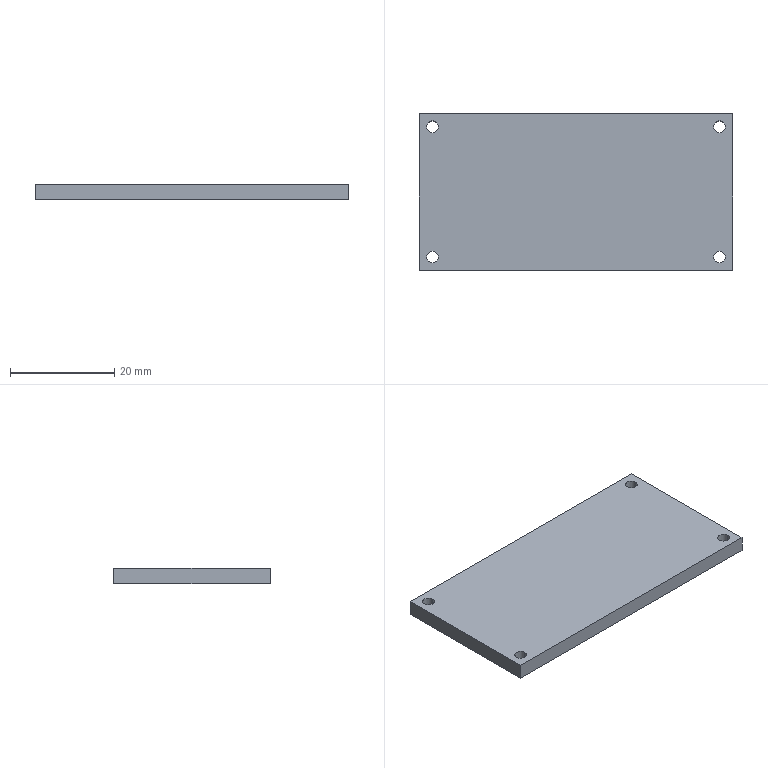Component | SolidWorks | Assembly3-1_Plate2555-1 | 1 solid | 14 faces | box 60 x 30 x 3 mm | volume 5353 mm3 | cylinder 8 | plane 6 | commonest cylinder face diameters 2.236 x8
build123d program:
from build123d import *

# Parameters (mm, degrees)
SKETCH1_W           = 60
SKETCH1_H           = 30
SKETCH1_R           = 1.118
BOSS_EXTRUDE1_DEPTH = 3


with BuildPart() as part:
    # Sketch1 → Boss-Extrude1 (new body)
    with BuildSketch(Plane.XY):
        Rectangle(SKETCH1_W, SKETCH1_H)
        with Locations((-27.5, 12.5)):
            Circle(SKETCH1_R, mode=Mode.SUBTRACT)
        with Locations(Location((27.5, 12.5, 0), (0, 0, 180))):
            Circle(SKETCH1_R, mode=Mode.SUBTRACT)
        with Locations((27.5, -12.5)):
            Circle(SKETCH1_R, mode=Mode.SUBTRACT)
        with Locations(Location((-27.5, -12.5, 0), (0, 0, 180))):
            Circle(SKETCH1_R, mode=Mode.SUBTRACT)
    extrude(amount=BOSS_EXTRUDE1_DEPTH)


solid = part.part

# Placed as in the assembly
solid = solid.moved(Location((0, -29.5, 38), (0, 0, 0)))
STEP:
#1=COLOUR_RGB('',0.7922,0.8196,0.9333);
#2=FILL_AREA_STYLE_COLOUR('',#1);
#3=FILL_AREA_STYLE('',(#2));
#4=SURFACE_STYLE_FILL_AREA(#3);
#5=SURFACE_SIDE_STYLE('',(#4));
#6=SURFACE_STYLE_USAGE(.BOTH.,#5);
#7=PRESENTATION_STYLE_ASSIGNMENT((#6));
#8=CARTESIAN_POINT('',(-1.127,-0.6693,1.496));
#9=VERTEX_POINT('',#8);
#10=CARTESIAN_POINT('',(-1.039,-0.6693,1.496));
#11=VERTEX_POINT('',#10);
#12=CARTESIAN_POINT('',(-1.083,-0.6693,1.496));
#13=DIRECTION('',(-0.,-0.,-1.));
#14=DIRECTION('',(-1.,0.,0.));
#15=AXIS2_PLACEMENT_3D('',#12,#13,#14);
#16=CIRCLE('',#15,0.04402);
#17=EDGE_CURVE('',#9,#11,#16,.T.);
#18=ORIENTED_EDGE('',*,*,#17,.T.);
#19=CARTESIAN_POINT('',(-1.039,-0.6693,1.614));
#20=VERTEX_POINT('',#19);
#21=CARTESIAN_POINT('',(-1.039,-0.6693,1.496));
#22=DIRECTION('',(0.,0.,1.));
#23=VECTOR('',#22,39.37);
#24=LINE('',#21,#23);
#25=EDGE_CURVE('',#11,#20,#24,.T.);
#26=ORIENTED_EDGE('',*,*,#25,.T.);
#27=CARTESIAN_POINT('',(-1.127,-0.6693,1.614));
#28=VERTEX_POINT('',#27);
#29=CARTESIAN_POINT('',(-1.083,-0.6693,1.614));
#30=DIRECTION('',(-0.,-0.,-1.));
#31=DIRECTION('',(-1.,0.,0.));
#32=AXIS2_PLACEMENT_3D('',#29,#30,#31);
#33=CIRCLE('',#32,0.04402);
#34=EDGE_CURVE('',#28,#20,#33,.T.);
#35=ORIENTED_EDGE('',*,*,#34,.F.);
#36=CARTESIAN_POINT('',(-1.127,-0.6693,1.496));
#37=DIRECTION('',(0.,0.,1.));
#38=VECTOR('',#37,39.37);
#39=LINE('',#36,#38);
#40=EDGE_CURVE('',#9,#28,#39,.T.);
#41=ORIENTED_EDGE('',*,*,#40,.F.);
#42=EDGE_LOOP('',(#18,#26,#35,#41));
#43=FACE_OUTER_BOUND('',#42,.T.);
#44=CARTESIAN_POINT('',(-1.083,-0.6693,1.496));
#45=DIRECTION('',(0.,0.,1.));
#46=DIRECTION('',(-1.,0.,0.));
#47=AXIS2_PLACEMENT_3D('',#44,#45,#46);
#48=CYLINDRICAL_SURFACE('',#47,0.04402);
#49=ADVANCED_FACE('',(#43),#48,.F.);
#50=CARTESIAN_POINT('',(1.039,-0.6693,1.496));
#51=VERTEX_POINT('',#50);
#52=CARTESIAN_POINT('',(1.127,-0.6693,1.496));
#53=VERTEX_POINT('',#52);
#54=CARTESIAN_POINT('',(1.083,-0.6693,1.496));
#55=DIRECTION('',(-0.,-0.,-1.));
#56=DIRECTION('',(1.,0.,0.));
#57=AXIS2_PLACEMENT_3D('',#54,#55,#56);
#58=CIRCLE('',#57,0.04402);
#59=EDGE_CURVE('',#51,#53,#58,.T.);
#60=ORIENTED_EDGE('',*,*,#59,.T.);
#61=CARTESIAN_POINT('',(1.127,-0.6693,1.614));
#62=VERTEX_POINT('',#61);
#63=CARTESIAN_POINT('',(1.127,-0.6693,1.496));
#64=DIRECTION('',(0.,0.,1.));
#65=VECTOR('',#64,39.37);
#66=LINE('',#63,#65);
#67=EDGE_CURVE('',#53,#62,#66,.T.);
#68=ORIENTED_EDGE('',*,*,#67,.T.);
#69=CARTESIAN_POINT('',(1.039,-0.6693,1.614));
#70=VERTEX_POINT('',#69);
#71=CARTESIAN_POINT('',(1.083,-0.6693,1.614));
#72=DIRECTION('',(-0.,-0.,-1.));
#73=DIRECTION('',(1.,0.,0.));
#74=AXIS2_PLACEMENT_3D('',#71,#72,#73);
#75=CIRCLE('',#74,0.04402);
#76=EDGE_CURVE('',#70,#62,#75,.T.);
#77=ORIENTED_EDGE('',*,*,#76,.F.);
#78=CARTESIAN_POINT('',(1.039,-0.6693,1.496));
#79=DIRECTION('',(0.,0.,1.));
#80=VECTOR('',#79,39.37);
#81=LINE('',#78,#80);
#82=EDGE_CURVE('',#51,#70,#81,.T.);
#83=ORIENTED_EDGE('',*,*,#82,.F.);
#84=EDGE_LOOP('',(#60,#68,#77,#83));
#85=FACE_OUTER_BOUND('',#84,.T.);
#86=CARTESIAN_POINT('',(1.083,-0.6693,1.496));
#87=DIRECTION('',(0.,0.,1.));
#88=DIRECTION('',(-1.,0.,0.));
#89=AXIS2_PLACEMENT_3D('',#86,#87,#88);
#90=CYLINDRICAL_SURFACE('',#89,0.04402);
#91=ADVANCED_FACE('',(#85),#90,.F.);
#92=CARTESIAN_POINT('',(1.039,-1.654,1.496));
#93=VERTEX_POINT('',#92);
#94=CARTESIAN_POINT('',(1.127,-1.654,1.496));
#95=VERTEX_POINT('',#94);
#96=CARTESIAN_POINT('',(1.083,-1.654,1.496));
#97=DIRECTION('',(-0.,-0.,-1.));
#98=DIRECTION('',(-1.,0.,0.));
#99=AXIS2_PLACEMENT_3D('',#96,#97,#98);
#100=CIRCLE('',#99,0.04402);
#101=EDGE_CURVE('',#93,#95,#100,.T.);
#102=ORIENTED_EDGE('',*,*,#101,.T.);
#103=CARTESIAN_POINT('',(1.127,-1.654,1.614));
#104=VERTEX_POINT('',#103);
#105=CARTESIAN_POINT('',(1.127,-1.654,1.496));
#106=DIRECTION('',(0.,0.,1.));
#107=VECTOR('',#106,39.37);
#108=LINE('',#105,#107);
#109=EDGE_CURVE('',#95,#104,#108,.T.);
#110=ORIENTED_EDGE('',*,*,#109,.T.);
#111=CARTESIAN_POINT('',(1.039,-1.654,1.614));
#112=VERTEX_POINT('',#111);
#113=CARTESIAN_POINT('',(1.083,-1.654,1.614));
#114=DIRECTION('',(-0.,-0.,-1.));
#115=DIRECTION('',(-1.,0.,0.));
#116=AXIS2_PLACEMENT_3D('',#113,#114,#115);
#117=CIRCLE('',#116,0.04402);
#118=EDGE_CURVE('',#112,#104,#117,.T.);
#119=ORIENTED_EDGE('',*,*,#118,.F.);
#120=CARTESIAN_POINT('',(1.039,-1.654,1.496));
#121=DIRECTION('',(0.,0.,1.));
#122=VECTOR('',#121,39.37);
#123=LINE('',#120,#122);
#124=EDGE_CURVE('',#93,#112,#123,.T.);
#125=ORIENTED_EDGE('',*,*,#124,.F.);
#126=EDGE_LOOP('',(#102,#110,#119,#125));
#127=FACE_OUTER_BOUND('',#126,.T.);
#128=CARTESIAN_POINT('',(1.083,-1.654,1.496));
#129=DIRECTION('',(0.,0.,1.));
#130=DIRECTION('',(-1.,0.,0.));
#131=AXIS2_PLACEMENT_3D('',#128,#129,#130);
#132=CYLINDRICAL_SURFACE('',#131,0.04402);
#133=ADVANCED_FACE('',(#127),#132,.F.);
#134=CARTESIAN_POINT('',(-1.127,-1.654,1.496));
#135=VERTEX_POINT('',#134);
#136=CARTESIAN_POINT('',(-1.039,-1.654,1.496));
#137=VERTEX_POINT('',#136);
#138=CARTESIAN_POINT('',(-1.083,-1.654,1.496));
#139=DIRECTION('',(-0.,-0.,-1.));
#140=DIRECTION('',(1.,0.,0.));
#141=AXIS2_PLACEMENT_3D('',#138,#139,#140);
#142=CIRCLE('',#141,0.04402);
#143=EDGE_CURVE('',#135,#137,#142,.T.);
#144=ORIENTED_EDGE('',*,*,#143,.T.);
#145=CARTESIAN_POINT('',(-1.039,-1.654,1.614));
#146=VERTEX_POINT('',#145);
#147=CARTESIAN_POINT('',(-1.039,-1.654,1.496));
#148=DIRECTION('',(0.,0.,1.));
#149=VECTOR('',#148,39.37);
#150=LINE('',#147,#149);
#151=EDGE_CURVE('',#137,#146,#150,.T.);
#152=ORIENTED_EDGE('',*,*,#151,.T.);
#153=CARTESIAN_POINT('',(-1.127,-1.654,1.614));
#154=VERTEX_POINT('',#153);
#155=CARTESIAN_POINT('',(-1.083,-1.654,1.614));
#156=DIRECTION('',(-0.,-0.,-1.));
#157=DIRECTION('',(1.,0.,0.));
#158=AXIS2_PLACEMENT_3D('',#155,#156,#157);
#159=CIRCLE('',#158,0.04402);
#160=EDGE_CURVE('',#154,#146,#159,.T.);
#161=ORIENTED_EDGE('',*,*,#160,.F.);
#162=CARTESIAN_POINT('',(-1.127,-1.654,1.496));
#163=DIRECTION('',(0.,0.,1.));
#164=VECTOR('',#163,39.37);
#165=LINE('',#162,#164);
#166=EDGE_CURVE('',#135,#154,#165,.T.);
#167=ORIENTED_EDGE('',*,*,#166,.F.);
#168=EDGE_LOOP('',(#144,#152,#161,#167));
#169=FACE_OUTER_BOUND('',#168,.T.);
#170=CARTESIAN_POINT('',(-1.083,-1.654,1.496));
#171=DIRECTION('',(0.,0.,1.));
#172=DIRECTION('',(-1.,0.,0.));
#173=AXIS2_PLACEMENT_3D('',#170,#171,#172);
#174=CYLINDRICAL_SURFACE('',#173,0.04402);
#175=ADVANCED_FACE('',(#169),#174,.F.);
#176=CARTESIAN_POINT('',(1.181,-0.5709,1.496));
#177=VERTEX_POINT('',#176);
#178=CARTESIAN_POINT('',(1.181,-1.752,1.496));
#179=VERTEX_POINT('',#178);
#180=CARTESIAN_POINT('',(1.181,-0.5709,1.496));
#181=DIRECTION('',(0.,-1.,0.));
#182=VECTOR('',#181,39.37);
#183=LINE('',#180,#182);
#184=EDGE_CURVE('',#177,#179,#183,.T.);
#185=ORIENTED_EDGE('',*,*,#184,.T.);
#186=CARTESIAN_POINT('',(-1.181,-1.752,1.496));
#187=VERTEX_POINT('',#186);
#188=CARTESIAN_POINT('',(-1.181,-1.752,1.496));
#189=DIRECTION('',(-1.,-0.,0.));
#190=VECTOR('',#189,39.37);
#191=LINE('',#188,#190);
#192=EDGE_CURVE('',#179,#187,#191,.T.);
#193=ORIENTED_EDGE('',*,*,#192,.T.);
#194=CARTESIAN_POINT('',(-1.181,-0.5709,1.496));
#195=VERTEX_POINT('',#194);
#196=CARTESIAN_POINT('',(-1.181,-0.5709,1.496));
#197=DIRECTION('',(-0.,1.,-0.));
#198=VECTOR('',#197,39.37);
#199=LINE('',#196,#198);
#200=EDGE_CURVE('',#187,#195,#199,.T.);
#201=ORIENTED_EDGE('',*,*,#200,.T.);
#202=CARTESIAN_POINT('',(-1.181,-0.5709,1.496));
#203=DIRECTION('',(1.,0.,-0.));
#204=VECTOR('',#203,39.37);
#205=LINE('',#202,#204);
#206=EDGE_CURVE('',#195,#177,#205,.T.);
#207=ORIENTED_EDGE('',*,*,#206,.T.);
#208=EDGE_LOOP('',(#185,#193,#201,#207));
#209=FACE_OUTER_BOUND('',#208,.T.);
#210=ORIENTED_EDGE('',*,*,#143,.F.);
#211=CARTESIAN_POINT('',(-1.083,-1.654,1.496));
#212=DIRECTION('',(-0.,-0.,-1.));
#213=DIRECTION('',(1.,0.,0.));
#214=AXIS2_PLACEMENT_3D('',#211,#212,#213);
#215=CIRCLE('',#214,0.04402);
#216=EDGE_CURVE('',#137,#135,#215,.T.);
#217=ORIENTED_EDGE('',*,*,#216,.F.);
#218=EDGE_LOOP('',(#210,#217));
#219=FACE_BOUND('',#218,.T.);
#220=ORIENTED_EDGE('',*,*,#101,.F.);
#221=CARTESIAN_POINT('',(1.083,-1.654,1.496));
#222=DIRECTION('',(-0.,-0.,-1.));
#223=DIRECTION('',(-1.,0.,0.));
#224=AXIS2_PLACEMENT_3D('',#221,#222,#223);
#225=CIRCLE('',#224,0.04402);
#226=EDGE_CURVE('',#95,#93,#225,.T.);
#227=ORIENTED_EDGE('',*,*,#226,.F.);
#228=EDGE_LOOP('',(#220,#227));
#229=FACE_BOUND('',#228,.T.);
#230=ORIENTED_EDGE('',*,*,#59,.F.);
#231=CARTESIAN_POINT('',(1.083,-0.6693,1.496));
#232=DIRECTION('',(-0.,-0.,-1.));
#233=DIRECTION('',(1.,0.,0.));
#234=AXIS2_PLACEMENT_3D('',#231,#232,#233);
#235=CIRCLE('',#234,0.04402);
#236=EDGE_CURVE('',#53,#51,#235,.T.);
#237=ORIENTED_EDGE('',*,*,#236,.F.);
#238=EDGE_LOOP('',(#230,#237));
#239=FACE_BOUND('',#238,.T.);
#240=ORIENTED_EDGE('',*,*,#17,.F.);
#241=CARTESIAN_POINT('',(-1.083,-0.6693,1.496));
#242=DIRECTION('',(-0.,-0.,-1.));
#243=DIRECTION('',(-1.,0.,0.));
#244=AXIS2_PLACEMENT_3D('',#241,#242,#243);
#245=CIRCLE('',#244,0.04402);
#246=EDGE_CURVE('',#11,#9,#245,.T.);
#247=ORIENTED_EDGE('',*,*,#246,.F.);
#248=EDGE_LOOP('',(#240,#247));
#249=FACE_BOUND('',#248,.T.);
#250=CARTESIAN_POINT('',(0.,-1.161,1.496));
#251=DIRECTION('',(0.,0.,1.));
#252=DIRECTION('',(-1.,-0.,0.));
#253=AXIS2_PLACEMENT_3D('',#250,#251,#252);
#254=PLANE('',#253);
#255=ADVANCED_FACE('',(#209,#219,#229,#239,#249),#254,.F.);
#256=ORIENTED_EDGE('',*,*,#76,.T.);
#257=CARTESIAN_POINT('',(1.083,-0.6693,1.614));
#258=DIRECTION('',(-0.,-0.,-1.));
#259=DIRECTION('',(1.,0.,0.));
#260=AXIS2_PLACEMENT_3D('',#257,#258,#259);
#261=CIRCLE('',#260,0.04402);
#262=EDGE_CURVE('',#62,#70,#261,.T.);
#263=ORIENTED_EDGE('',*,*,#262,.T.);
#264=EDGE_LOOP('',(#256,#263));
#265=FACE_BOUND('',#264,.T.);
#266=ORIENTED_EDGE('',*,*,#160,.T.);
#267=CARTESIAN_POINT('',(-1.083,-1.654,1.614));
#268=DIRECTION('',(-0.,-0.,-1.));
#269=DIRECTION('',(1.,0.,0.));
#270=AXIS2_PLACEMENT_3D('',#267,#268,#269);
#271=CIRCLE('',#270,0.04402);
#272=EDGE_CURVE('',#146,#154,#271,.T.);
#273=ORIENTED_EDGE('',*,*,#272,.T.);
#274=EDGE_LOOP('',(#266,#273));
#275=FACE_BOUND('',#274,.T.);
#276=CARTESIAN_POINT('',(1.181,-0.5709,1.614));
#277=VERTEX_POINT('',#276);
#278=CARTESIAN_POINT('',(1.181,-1.752,1.614));
#279=VERTEX_POINT('',#278);
#280=CARTESIAN_POINT('',(1.181,-0.5709,1.614));
#281=DIRECTION('',(0.,-1.,0.));
#282=VECTOR('',#281,39.37);
#283=LINE('',#280,#282);
#284=EDGE_CURVE('',#277,#279,#283,.T.);
#285=ORIENTED_EDGE('',*,*,#284,.F.);
#286=CARTESIAN_POINT('',(-1.181,-0.5709,1.614));
#287=VERTEX_POINT('',#286);
#288=CARTESIAN_POINT('',(-1.181,-0.5709,1.614));
#289=DIRECTION('',(1.,0.,-0.));
#290=VECTOR('',#289,39.37);
#291=LINE('',#288,#290);
#292=EDGE_CURVE('',#287,#277,#291,.T.);
#293=ORIENTED_EDGE('',*,*,#292,.F.);
#294=CARTESIAN_POINT('',(-1.181,-1.752,1.614));
#295=VERTEX_POINT('',#294);
#296=CARTESIAN_POINT('',(-1.181,-0.5709,1.614));
#297=DIRECTION('',(-0.,1.,-0.));
#298=VECTOR('',#297,39.37);
#299=LINE('',#296,#298);
#300=EDGE_CURVE('',#295,#287,#299,.T.);
#301=ORIENTED_EDGE('',*,*,#300,.F.);
#302=CARTESIAN_POINT('',(-1.181,-1.752,1.614));
#303=DIRECTION('',(-1.,-0.,0.));
#304=VECTOR('',#303,39.37);
#305=LINE('',#302,#304);
#306=EDGE_CURVE('',#279,#295,#305,.T.);
#307=ORIENTED_EDGE('',*,*,#306,.F.);
#308=EDGE_LOOP('',(#285,#293,#301,#307));
#309=FACE_OUTER_BOUND('',#308,.T.);
#310=ORIENTED_EDGE('',*,*,#118,.T.);
#311=CARTESIAN_POINT('',(1.083,-1.654,1.614));
#312=DIRECTION('',(-0.,-0.,-1.));
#313=DIRECTION('',(-1.,0.,0.));
#314=AXIS2_PLACEMENT_3D('',#311,#312,#313);
#315=CIRCLE('',#314,0.04402);
#316=EDGE_CURVE('',#104,#112,#315,.T.);
#317=ORIENTED_EDGE('',*,*,#316,.T.);
#318=EDGE_LOOP('',(#310,#317));
#319=FACE_BOUND('',#318,.T.);
#320=ORIENTED_EDGE('',*,*,#34,.T.);
#321=CARTESIAN_POINT('',(-1.083,-0.6693,1.614));
#322=DIRECTION('',(-0.,-0.,-1.));
#323=DIRECTION('',(-1.,0.,0.));
#324=AXIS2_PLACEMENT_3D('',#321,#322,#323);
#325=CIRCLE('',#324,0.04402);
#326=EDGE_CURVE('',#20,#28,#325,.T.);
#327=ORIENTED_EDGE('',*,*,#326,.T.);
#328=EDGE_LOOP('',(#320,#327));
#329=FACE_BOUND('',#328,.T.);
#330=CARTESIAN_POINT('',(0.,-1.161,1.614));
#331=DIRECTION('',(0.,0.,1.));
#332=DIRECTION('',(-1.,-0.,0.));
#333=AXIS2_PLACEMENT_3D('',#330,#331,#332);
#334=PLANE('',#333);
#335=ADVANCED_FACE('',(#265,#275,#309,#319,#329),#334,.T.);
#336=ORIENTED_EDGE('',*,*,#284,.T.);
#337=CARTESIAN_POINT('',(1.181,-1.752,1.496));
#338=DIRECTION('',(0.,0.,1.));
#339=VECTOR('',#338,39.37);
#340=LINE('',#337,#339);
#341=EDGE_CURVE('',#179,#279,#340,.T.);
#342=ORIENTED_EDGE('',*,*,#341,.F.);
#343=ORIENTED_EDGE('',*,*,#184,.F.);
#344=CARTESIAN_POINT('',(1.181,-0.5709,1.496));
#345=DIRECTION('',(0.,0.,1.));
#346=VECTOR('',#345,39.37);
#347=LINE('',#344,#346);
#348=EDGE_CURVE('',#177,#277,#347,.T.);
#349=ORIENTED_EDGE('',*,*,#348,.T.);
#350=EDGE_LOOP('',(#336,#342,#343,#349));
#351=FACE_OUTER_BOUND('',#350,.T.);
#352=CARTESIAN_POINT('',(1.181,-0.5709,1.496));
#353=DIRECTION('',(-1.,-0.,0.));
#354=DIRECTION('',(-0.,-0.,-1.));
#355=AXIS2_PLACEMENT_3D('',#352,#353,#354);
#356=PLANE('',#355);
#357=ADVANCED_FACE('',(#351),#356,.F.);
#358=ORIENTED_EDGE('',*,*,#306,.T.);
#359=CARTESIAN_POINT('',(-1.181,-1.752,1.496));
#360=DIRECTION('',(0.,0.,1.));
#361=VECTOR('',#360,39.37);
#362=LINE('',#359,#361);
#363=EDGE_CURVE('',#187,#295,#362,.T.);
#364=ORIENTED_EDGE('',*,*,#363,.F.);
#365=ORIENTED_EDGE('',*,*,#192,.F.);
#366=ORIENTED_EDGE('',*,*,#341,.T.);
#367=EDGE_LOOP('',(#358,#364,#365,#366));
#368=FACE_OUTER_BOUND('',#367,.T.);
#369=CARTESIAN_POINT('',(-1.181,-1.752,1.496));
#370=DIRECTION('',(-0.,1.,-0.));
#371=DIRECTION('',(0.,0.,1.));
#372=AXIS2_PLACEMENT_3D('',#369,#370,#371);
#373=PLANE('',#372);
#374=ADVANCED_FACE('',(#368),#373,.F.);
#375=ORIENTED_EDGE('',*,*,#300,.T.);
#376=CARTESIAN_POINT('',(-1.181,-0.5709,1.496));
#377=DIRECTION('',(0.,0.,1.));
#378=VECTOR('',#377,39.37);
#379=LINE('',#376,#378);
#380=EDGE_CURVE('',#195,#287,#379,.T.);
#381=ORIENTED_EDGE('',*,*,#380,.F.);
#382=ORIENTED_EDGE('',*,*,#200,.F.);
#383=ORIENTED_EDGE('',*,*,#363,.T.);
#384=EDGE_LOOP('',(#375,#381,#382,#383));
#385=FACE_OUTER_BOUND('',#384,.T.);
#386=CARTESIAN_POINT('',(-1.181,-0.5709,1.496));
#387=DIRECTION('',(1.,0.,-0.));
#388=DIRECTION('',(0.,0.,1.));
#389=AXIS2_PLACEMENT_3D('',#386,#387,#388);
#390=PLANE('',#389);
#391=ADVANCED_FACE('',(#385),#390,.F.);
#392=ORIENTED_EDGE('',*,*,#292,.T.);
#393=ORIENTED_EDGE('',*,*,#348,.F.);
#394=ORIENTED_EDGE('',*,*,#206,.F.);
#395=ORIENTED_EDGE('',*,*,#380,.T.);
#396=EDGE_LOOP('',(#392,#393,#394,#395));
#397=FACE_OUTER_BOUND('',#396,.T.);
#398=CARTESIAN_POINT('',(-1.181,-0.5709,1.496));
#399=DIRECTION('',(0.,-1.,0.));
#400=DIRECTION('',(-0.,-0.,-1.));
#401=AXIS2_PLACEMENT_3D('',#398,#399,#400);
#402=PLANE('',#401);
#403=ADVANCED_FACE('',(#397),#402,.F.);
#404=ORIENTED_EDGE('',*,*,#151,.F.);
#405=ORIENTED_EDGE('',*,*,#216,.T.);
#406=ORIENTED_EDGE('',*,*,#166,.T.);
#407=ORIENTED_EDGE('',*,*,#272,.F.);
#408=EDGE_LOOP('',(#404,#405,#406,#407));
#409=FACE_OUTER_BOUND('',#408,.T.);
#410=CARTESIAN_POINT('',(-1.083,-1.654,1.496));
#411=DIRECTION('',(0.,0.,1.));
#412=DIRECTION('',(-1.,0.,0.));
#413=AXIS2_PLACEMENT_3D('',#410,#411,#412);
#414=CYLINDRICAL_SURFACE('',#413,0.04402);
#415=ADVANCED_FACE('',(#409),#414,.F.);
#416=ORIENTED_EDGE('',*,*,#109,.F.);
#417=ORIENTED_EDGE('',*,*,#226,.T.);
#418=ORIENTED_EDGE('',*,*,#124,.T.);
#419=ORIENTED_EDGE('',*,*,#316,.F.);
#420=EDGE_LOOP('',(#416,#417,#418,#419));
#421=FACE_OUTER_BOUND('',#420,.T.);
#422=CARTESIAN_POINT('',(1.083,-1.654,1.496));
#423=DIRECTION('',(0.,0.,1.));
#424=DIRECTION('',(-1.,0.,0.));
#425=AXIS2_PLACEMENT_3D('',#422,#423,#424);
#426=CYLINDRICAL_SURFACE('',#425,0.04402);
#427=ADVANCED_FACE('',(#421),#426,.F.);
#428=ORIENTED_EDGE('',*,*,#67,.F.);
#429=ORIENTED_EDGE('',*,*,#236,.T.);
#430=ORIENTED_EDGE('',*,*,#82,.T.);
#431=ORIENTED_EDGE('',*,*,#262,.F.);
#432=EDGE_LOOP('',(#428,#429,#430,#431));
#433=FACE_OUTER_BOUND('',#432,.T.);
#434=CARTESIAN_POINT('',(1.083,-0.6693,1.496));
#435=DIRECTION('',(0.,0.,1.));
#436=DIRECTION('',(-1.,0.,0.));
#437=AXIS2_PLACEMENT_3D('',#434,#435,#436);
#438=CYLINDRICAL_SURFACE('',#437,0.04402);
#439=ADVANCED_FACE('',(#433),#438,.F.);
#440=ORIENTED_EDGE('',*,*,#25,.F.);
#441=ORIENTED_EDGE('',*,*,#246,.T.);
#442=ORIENTED_EDGE('',*,*,#40,.T.);
#443=ORIENTED_EDGE('',*,*,#326,.F.);
#444=EDGE_LOOP('',(#440,#441,#442,#443));
#445=FACE_OUTER_BOUND('',#444,.T.);
#446=CARTESIAN_POINT('',(-1.083,-0.6693,1.496));
#447=DIRECTION('',(0.,0.,1.));
#448=DIRECTION('',(-1.,0.,0.));
#449=AXIS2_PLACEMENT_3D('',#446,#447,#448);
#450=CYLINDRICAL_SURFACE('',#449,0.04402);
#451=ADVANCED_FACE('',(#445),#450,.F.);
#452=CLOSED_SHELL('',(#49,#91,#133,#175,#255,#335,#357,#374,#391,#403,#415,#427,#439,#451));
#453=MANIFOLD_SOLID_BREP('',#452);
#454=STYLED_ITEM('',(#7),#453);
#455=PRESENTATION_LAYER_ASSIGNMENT('','',(#454));
#456=(LENGTH_UNIT()NAMED_UNIT(*)SI_UNIT($,.METRE.));
#457=LENGTH_MEASURE_WITH_UNIT(LENGTH_MEASURE(0.0254),#456);
#458=DIMENSIONAL_EXPONENTS(1.,0.,0.,0.,0.,0.,0.);
#459=(CONVERSION_BASED_UNIT('',#457)LENGTH_UNIT()NAMED_UNIT(#458));
#460=UNCERTAINTY_MEASURE_WITH_UNIT(LENGTH_MEASURE(0.00001),#459,'','');
#461=(NAMED_UNIT(*)PLANE_ANGLE_UNIT()SI_UNIT($,.RADIAN.));
#462=(NAMED_UNIT(*)SI_UNIT($,.STERADIAN.)SOLID_ANGLE_UNIT());
#463=(GEOMETRIC_REPRESENTATION_CONTEXT(3)GLOBAL_UNCERTAINTY_ASSIGNED_CONTEXT((#460))GLOBAL_UNIT_ASSIGNED_CONTEXT((#459,#461,#462))REPRESENTATION_CONTEXT('',''));
#464=MECHANICAL_DESIGN_GEOMETRIC_PRESENTATION_REPRESENTATION('',(#454),#463);
#465=CARTESIAN_POINT('',(0.,0.,0.));
#466=DIRECTION('',(0.,0.,1.));
#467=DIRECTION('',(1.,0.,0.));
#468=AXIS2_PLACEMENT_3D('',#465,#466,#467);
#469=(LENGTH_UNIT()NAMED_UNIT(*)SI_UNIT($,.METRE.));
#470=LENGTH_MEASURE_WITH_UNIT(LENGTH_MEASURE(0.0254),#469);
#471=DIMENSIONAL_EXPONENTS(1.,0.,0.,0.,0.,0.,0.);
#472=(CONVERSION_BASED_UNIT('',#470)LENGTH_UNIT()NAMED_UNIT(#471));
#473=UNCERTAINTY_MEASURE_WITH_UNIT(LENGTH_MEASURE(0.00001),#472,'','');
#474=(NAMED_UNIT(*)PLANE_ANGLE_UNIT()SI_UNIT($,.RADIAN.));
#475=(NAMED_UNIT(*)SI_UNIT($,.STERADIAN.)SOLID_ANGLE_UNIT());
#476=(GEOMETRIC_REPRESENTATION_CONTEXT(3)GLOBAL_UNCERTAINTY_ASSIGNED_CONTEXT((#473))GLOBAL_UNIT_ASSIGNED_CONTEXT((#472,#474,#475))REPRESENTATION_CONTEXT('',''));
#477=ADVANCED_BREP_SHAPE_REPRESENTATION('',(#453,#468),#476);